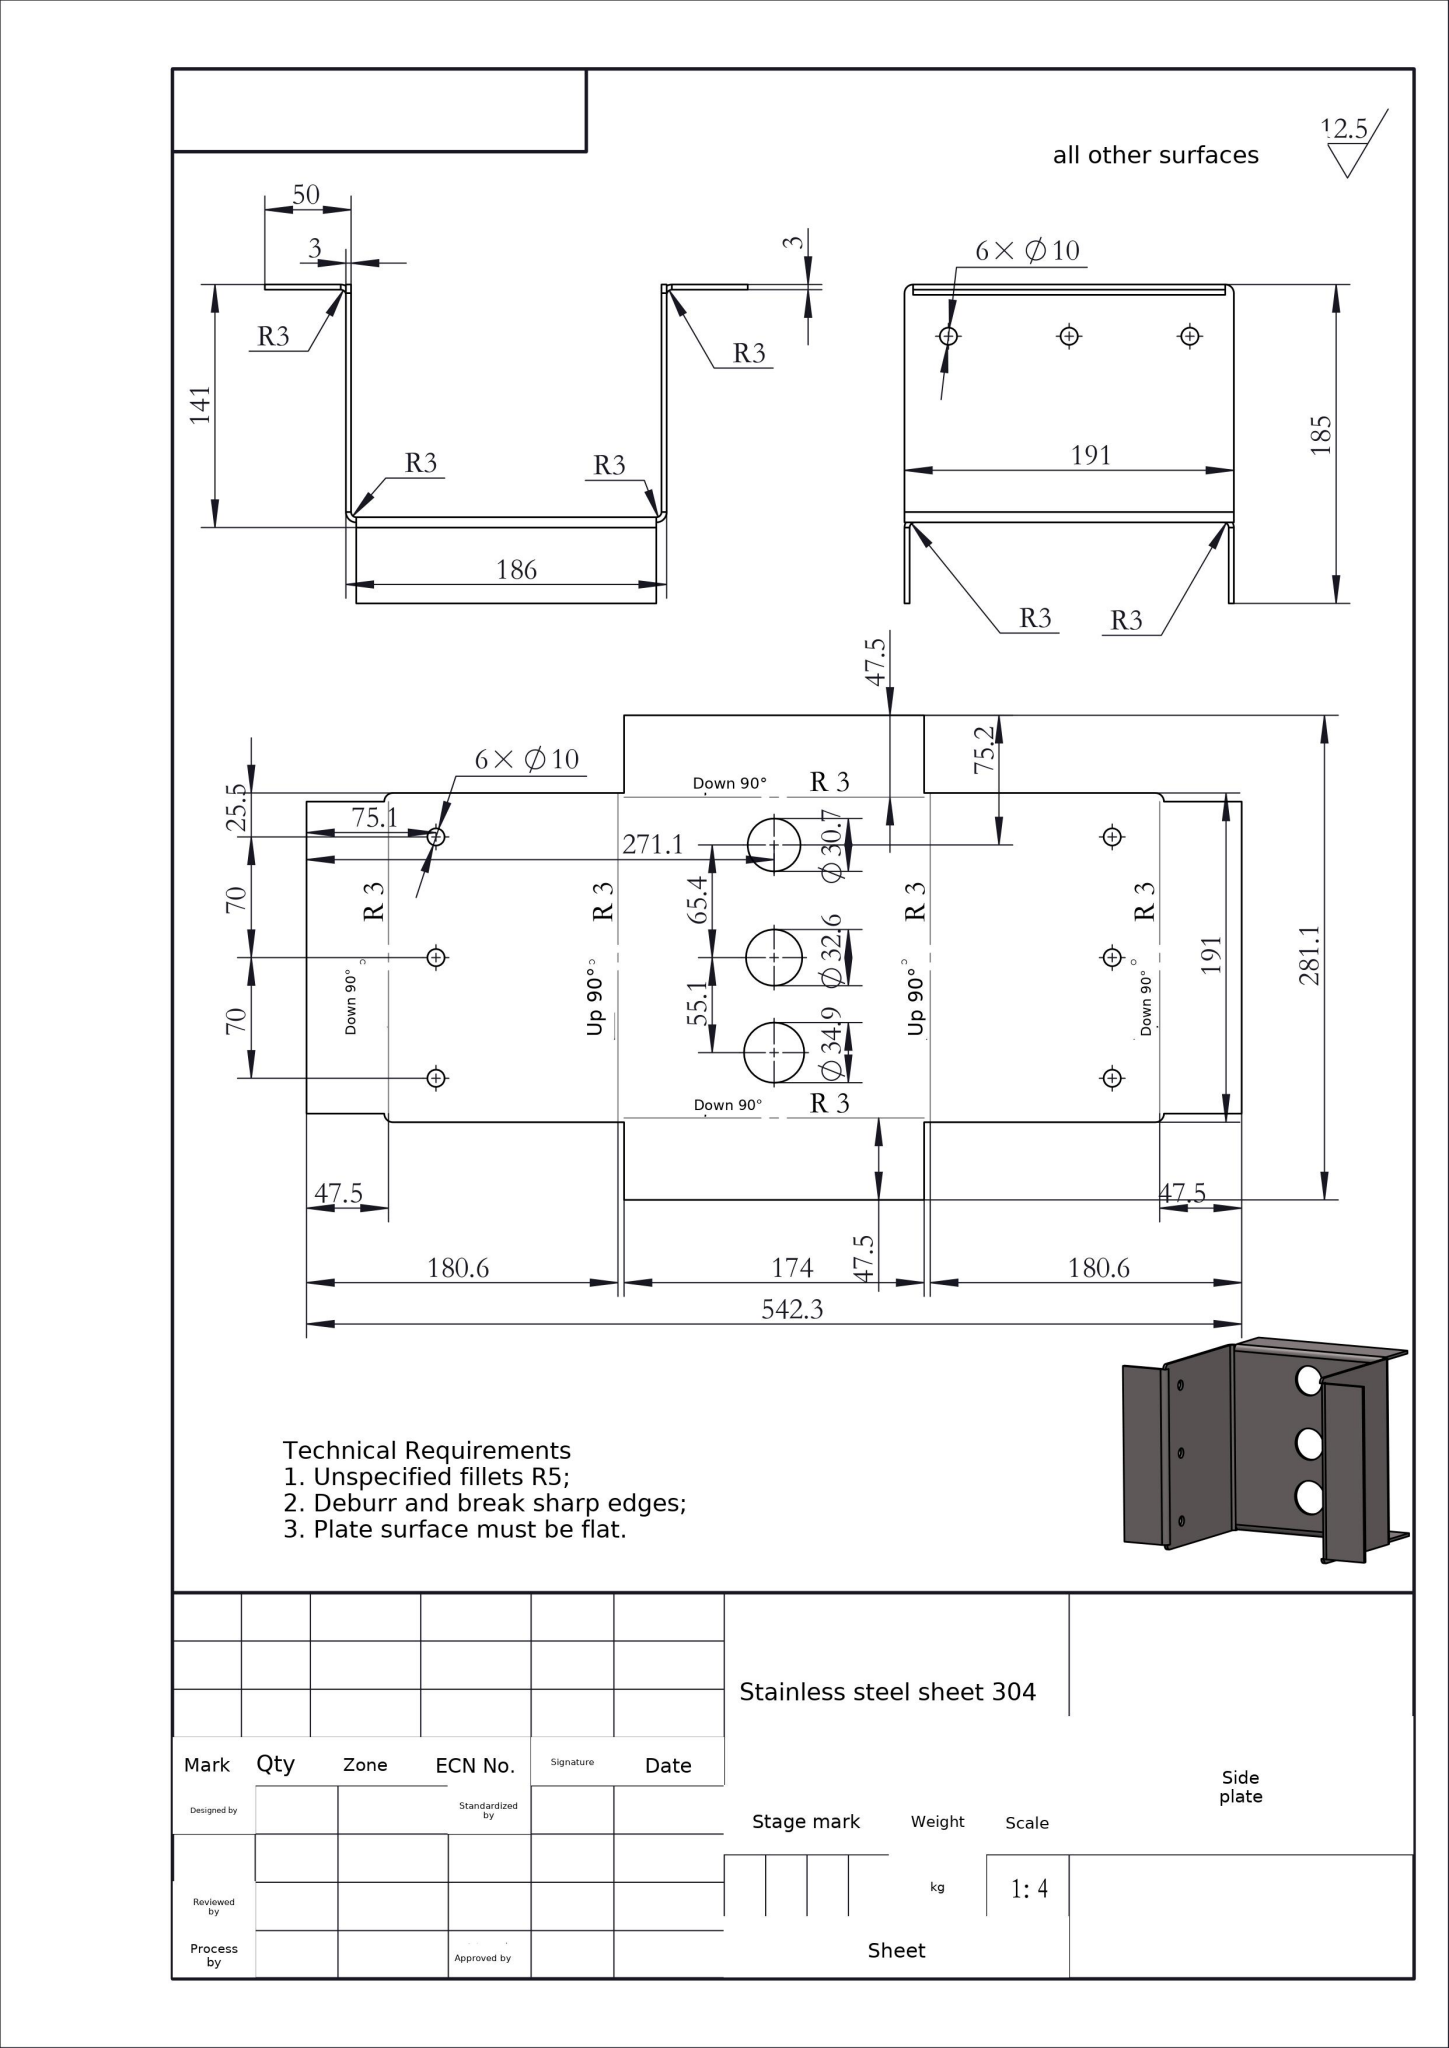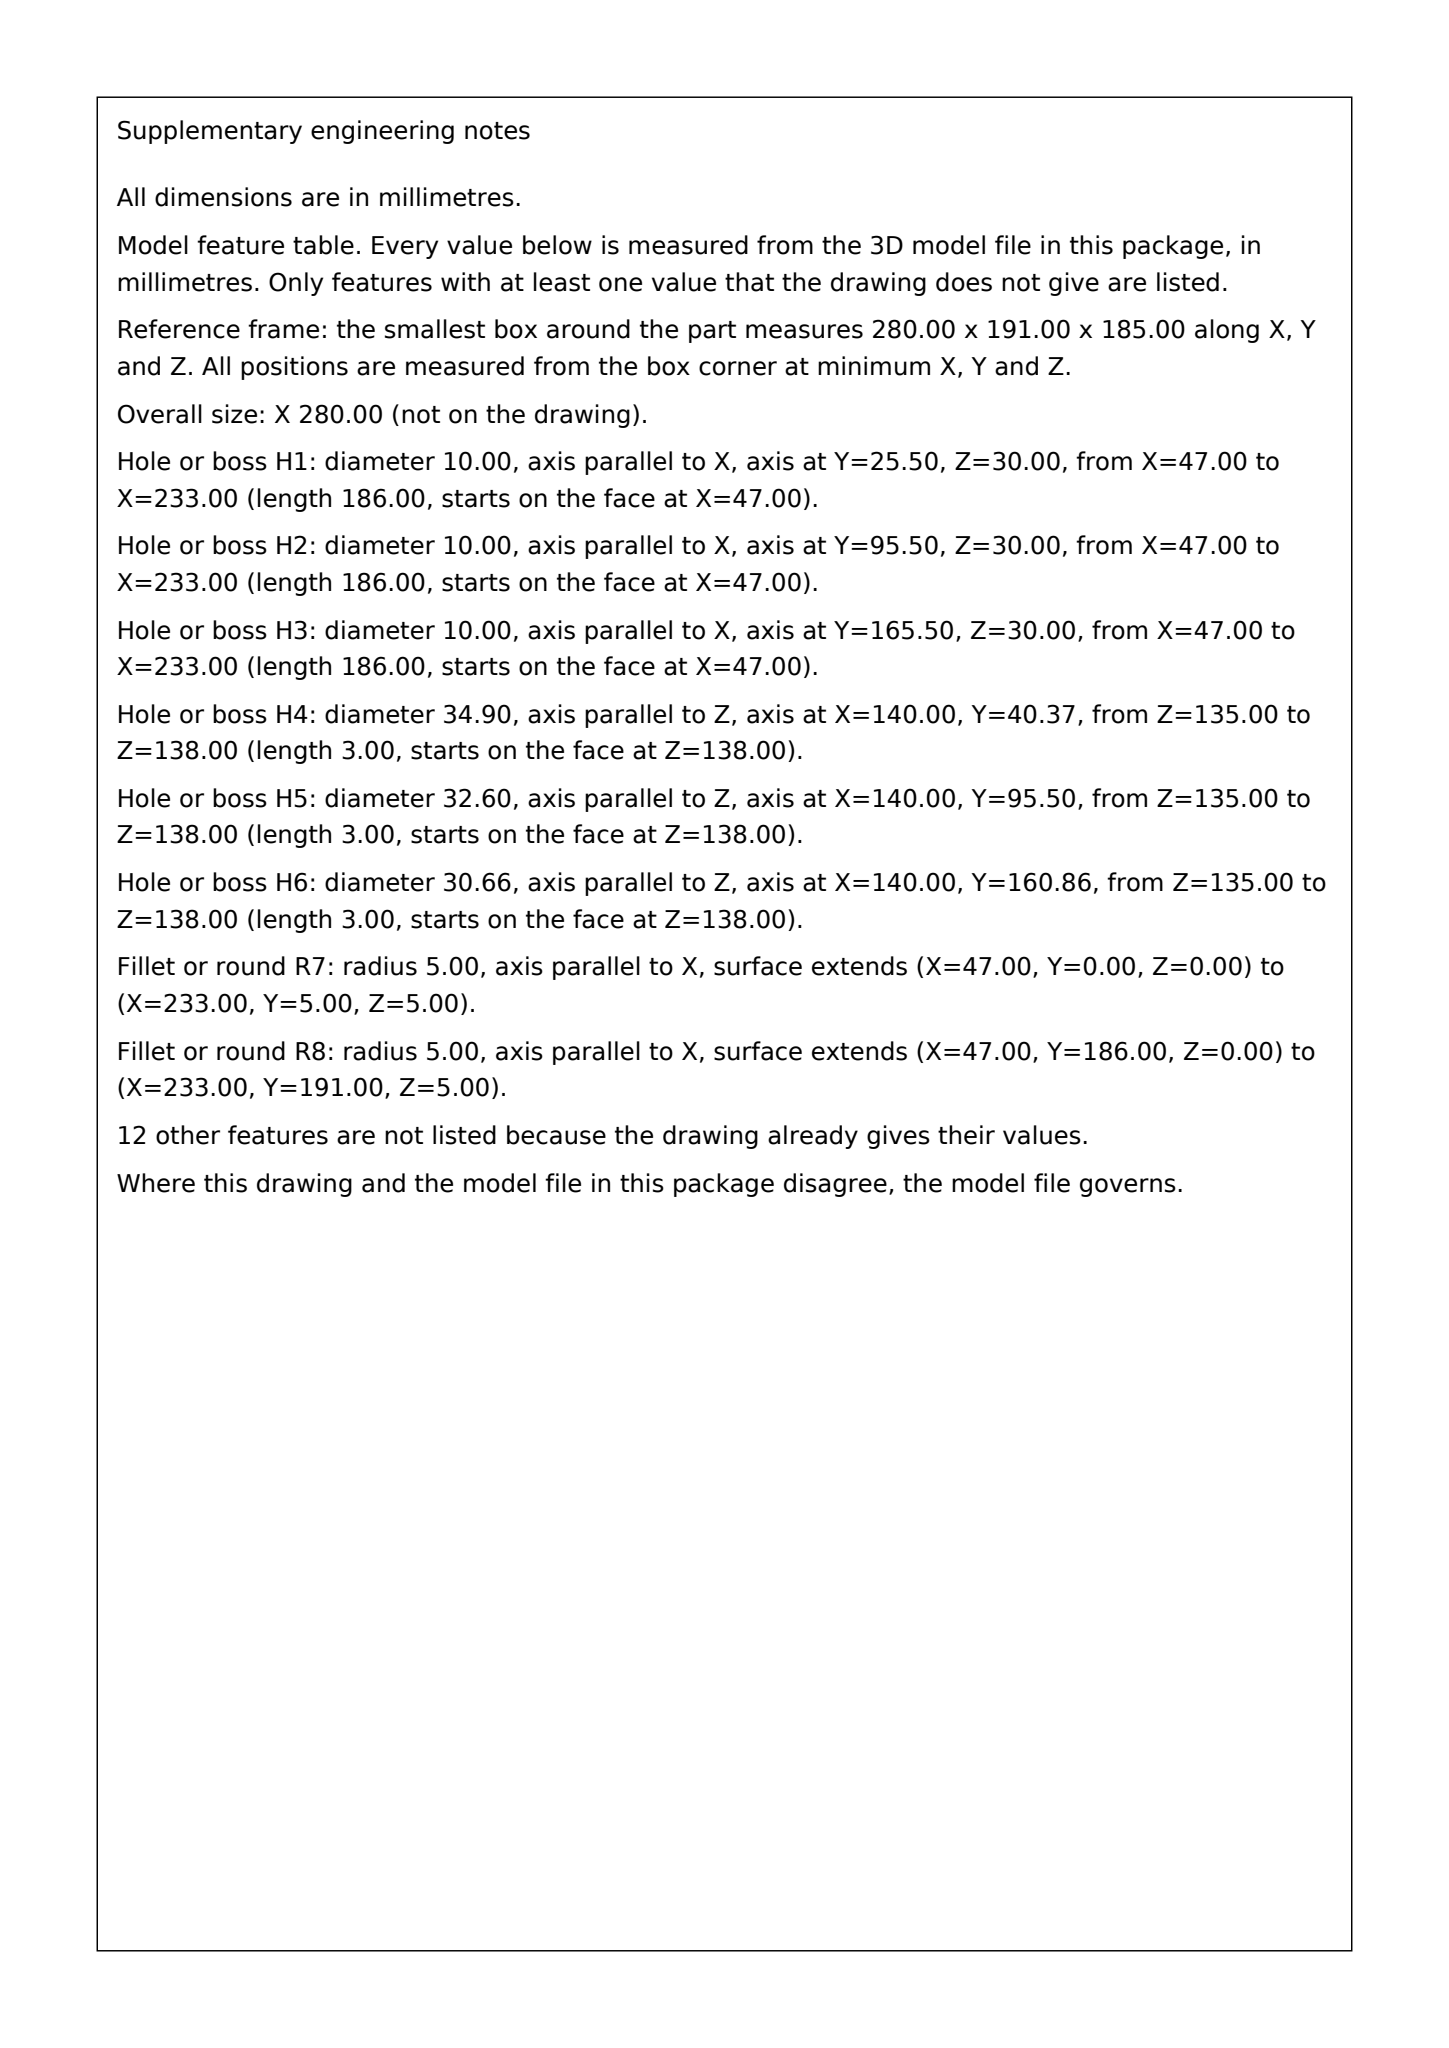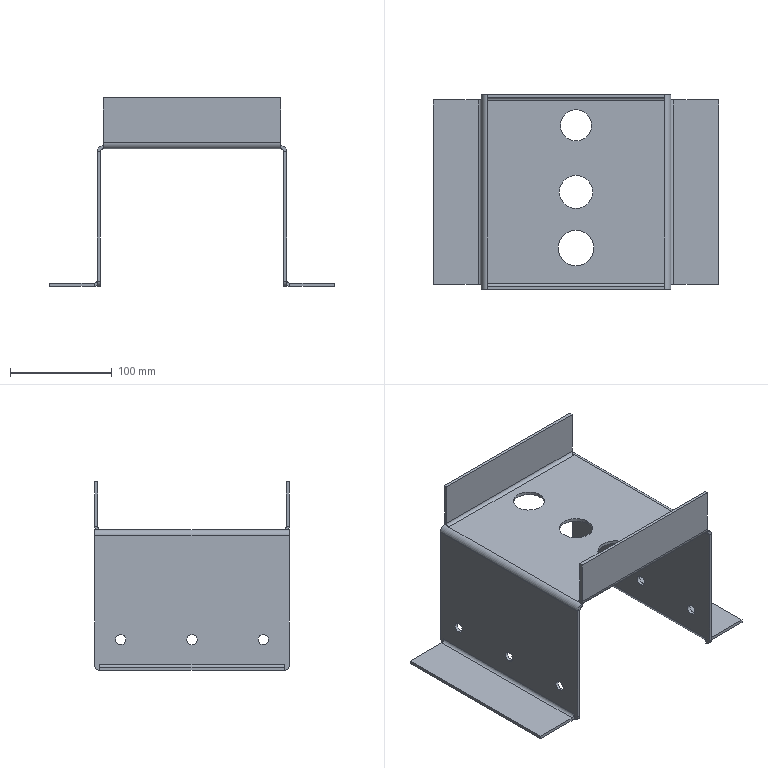Part | SolidWorks | mm | material Stainless steel sheet 304 | 1 solid | 84 faces | box 280 x 191 x 185 mm | volume 346005 mm3 | plane 50 | cylinder 34 | commonest cylinder face diameters 10 x16 12 x6 6 x6 30.66 x2 32.605 x2 34.891 x2